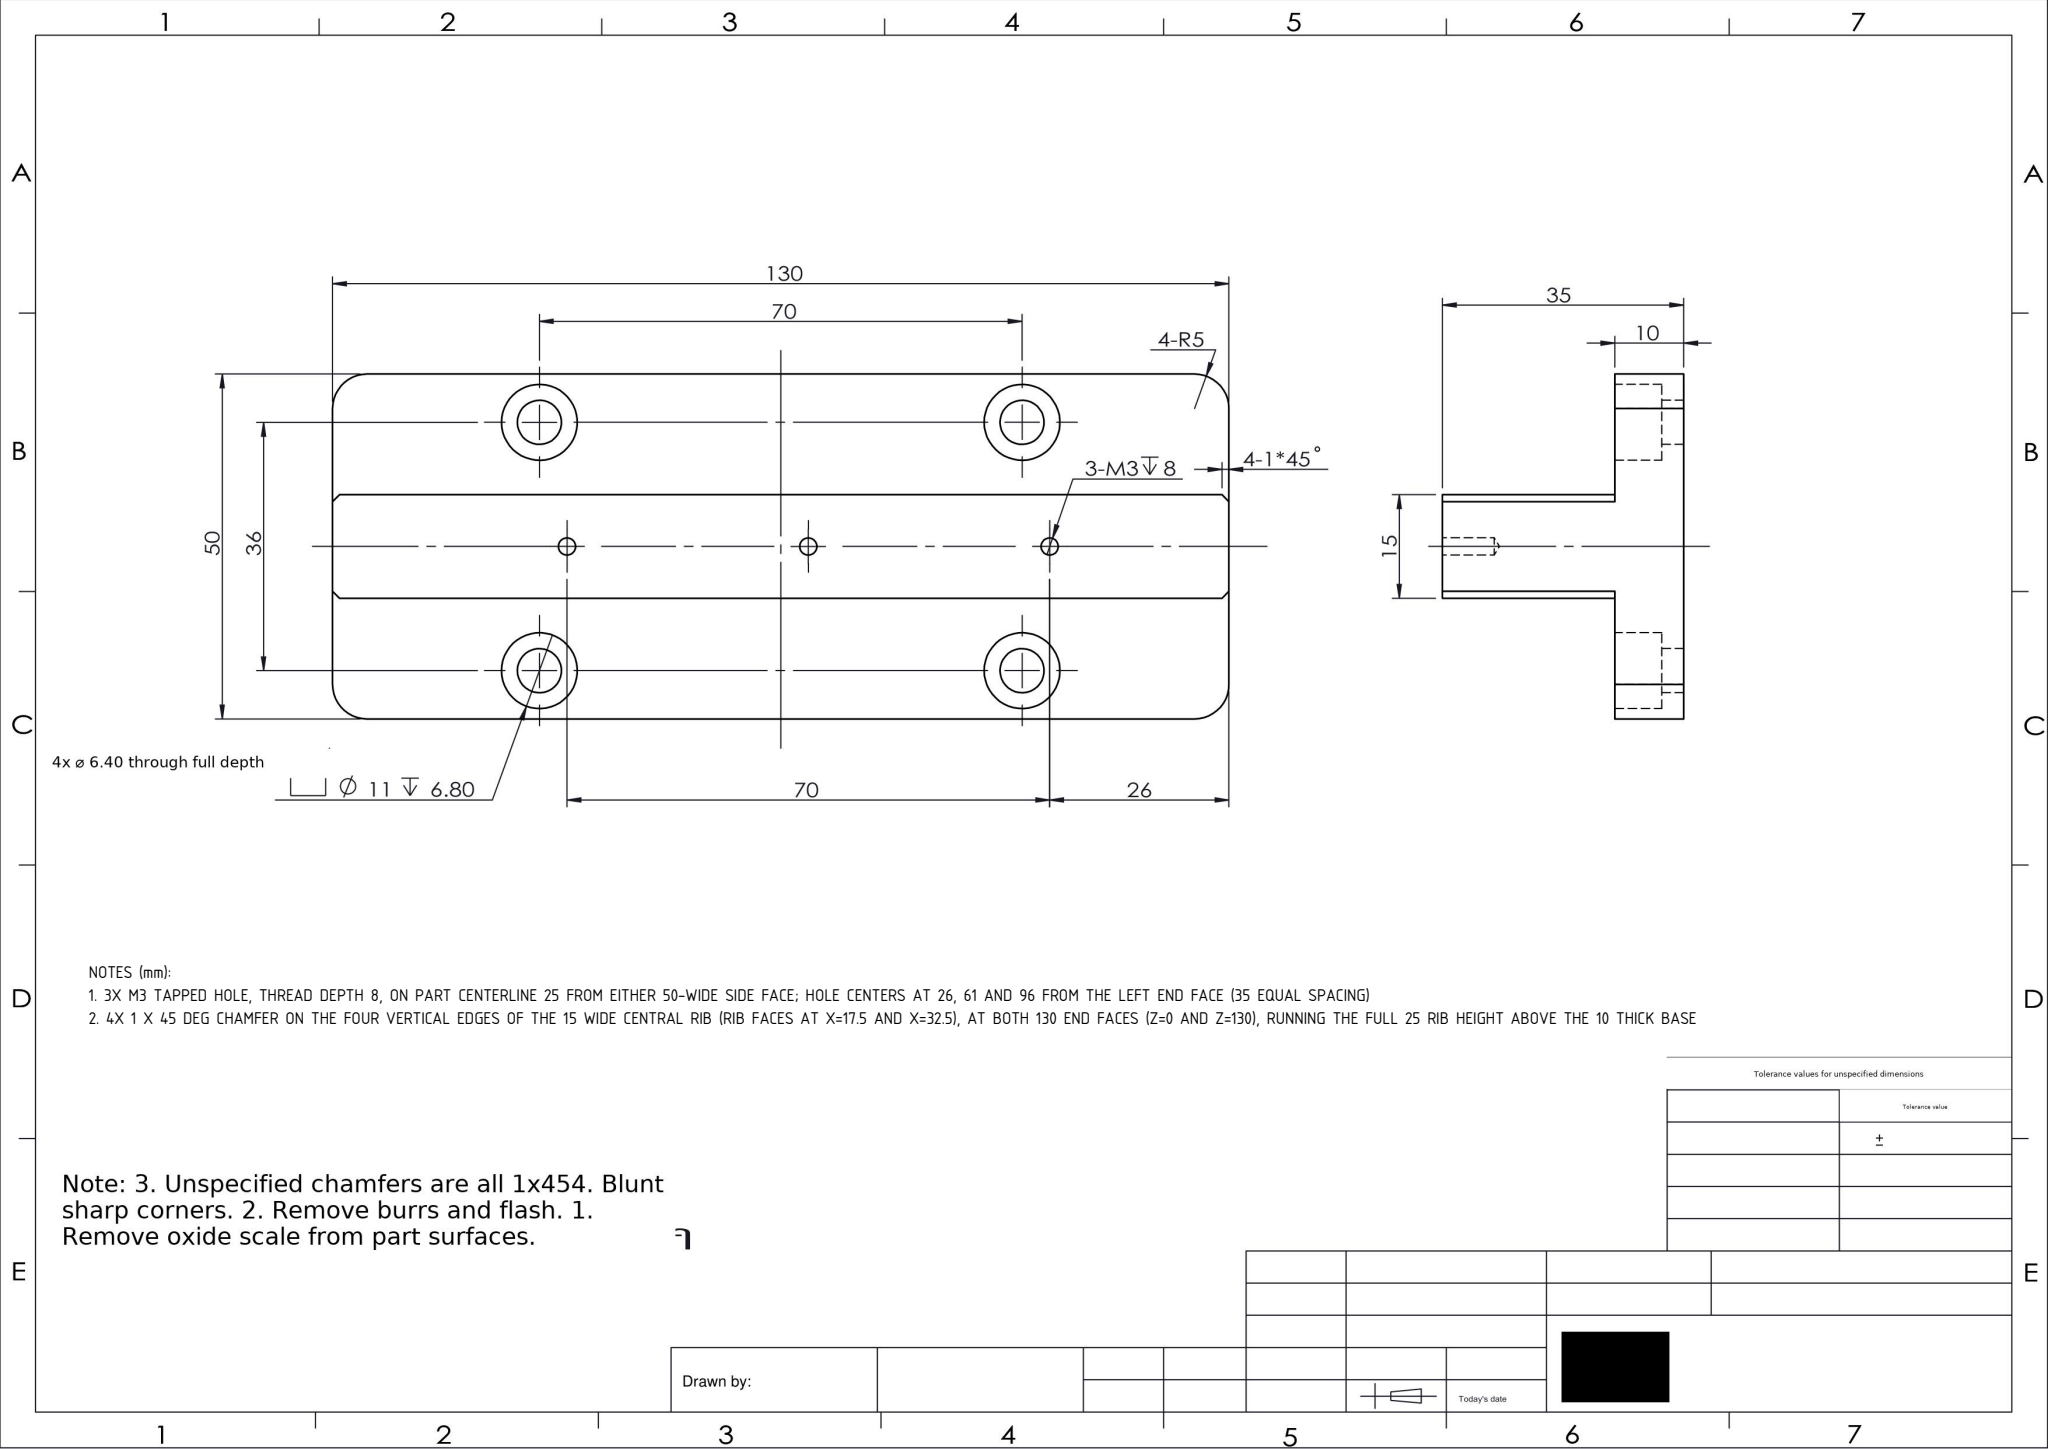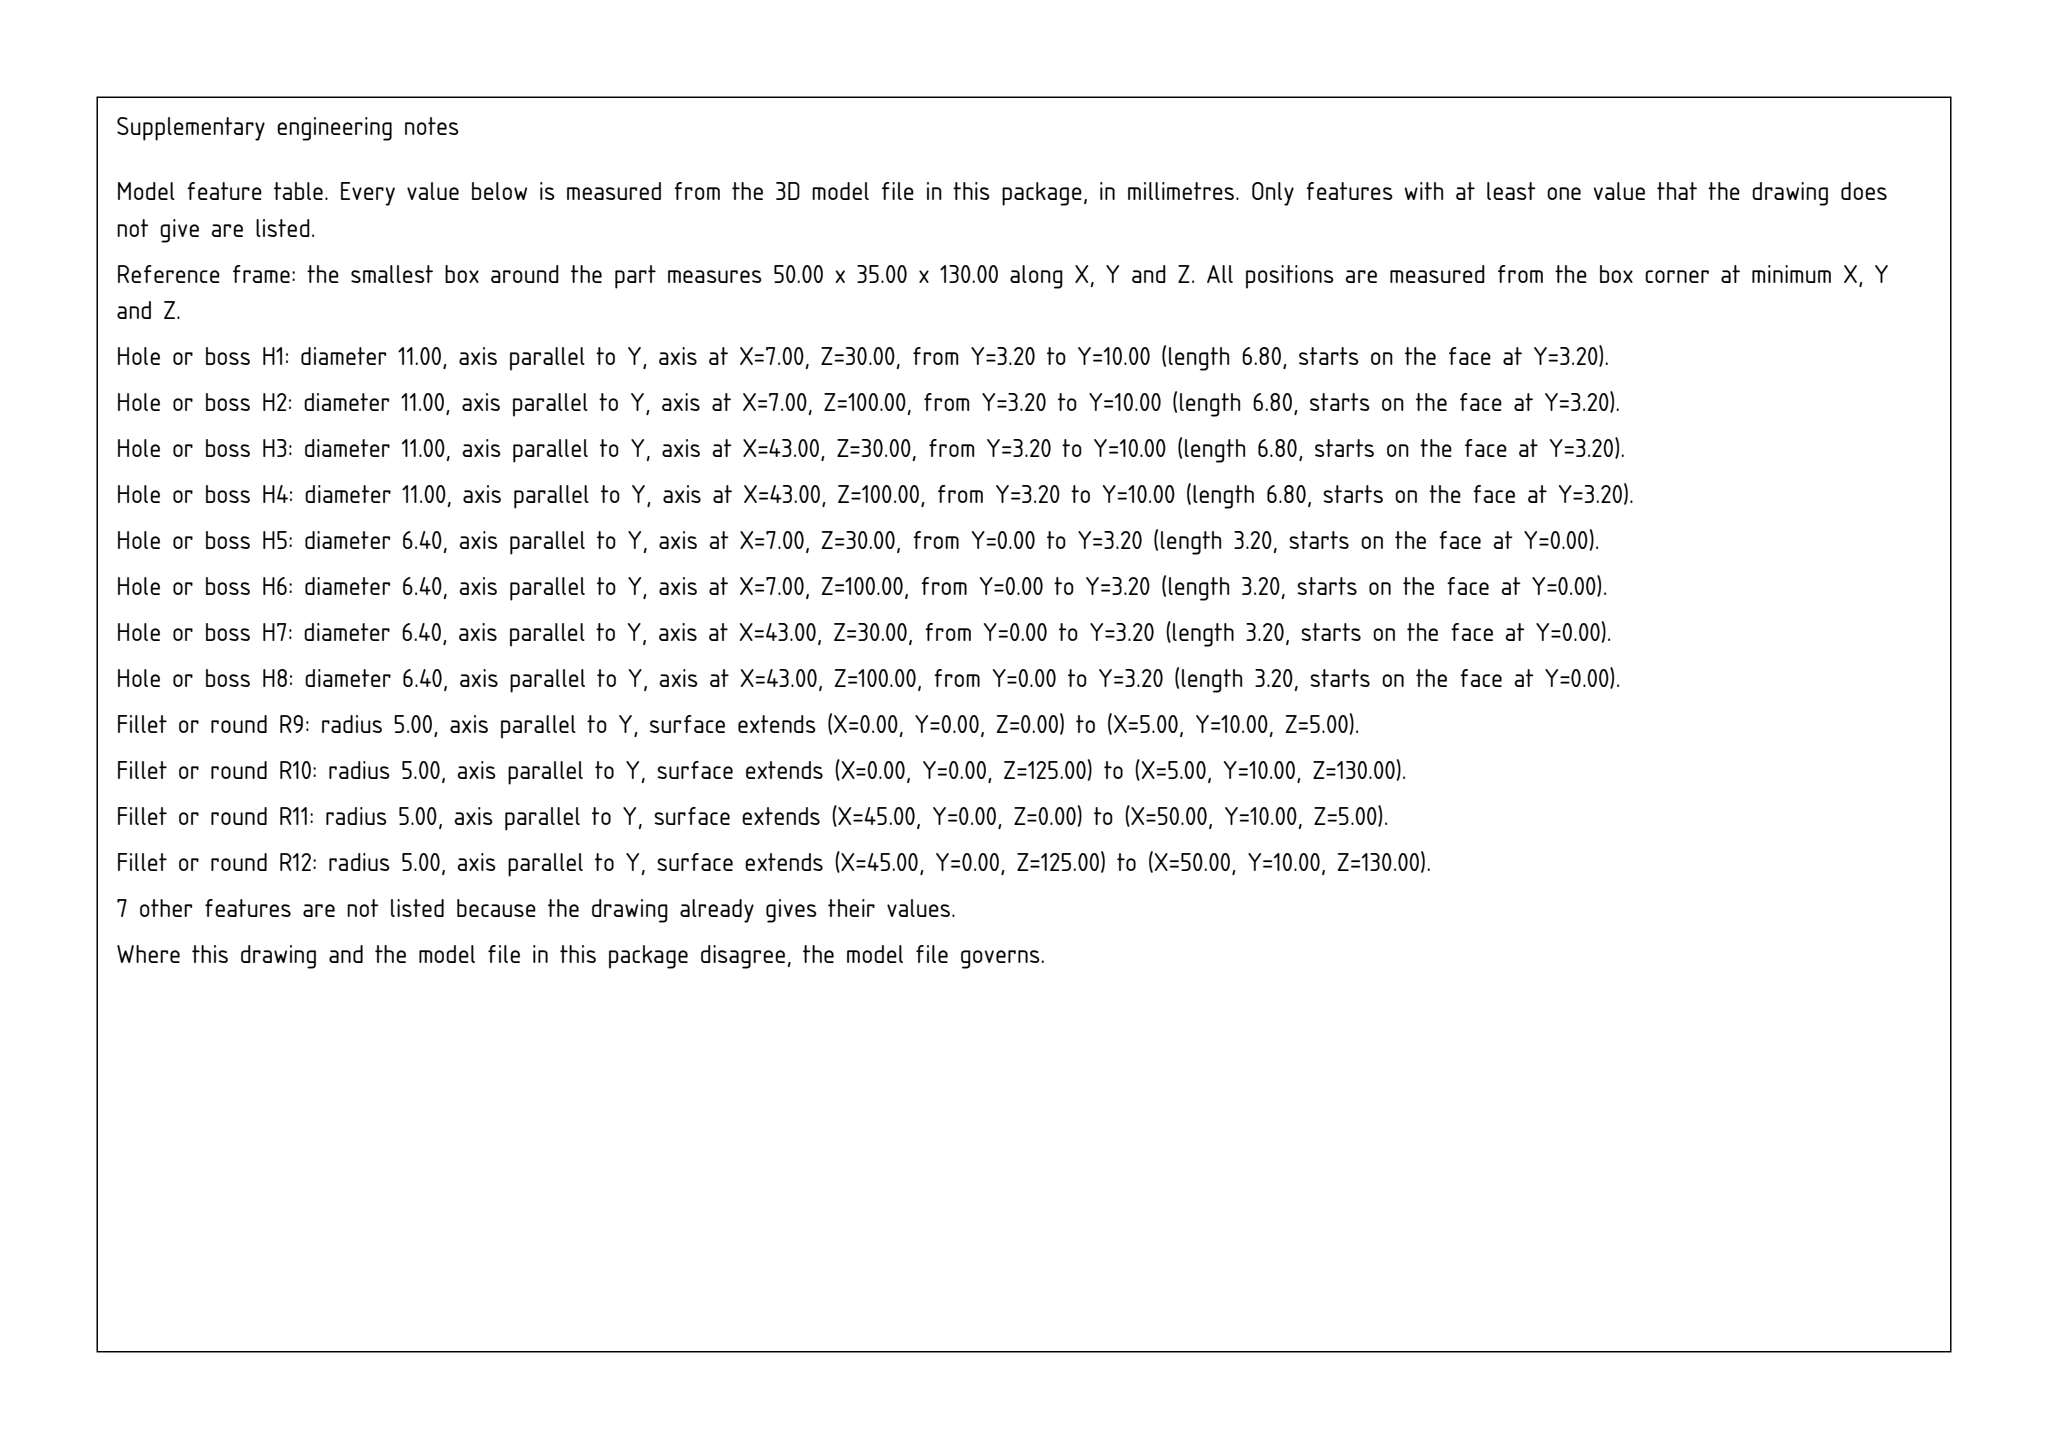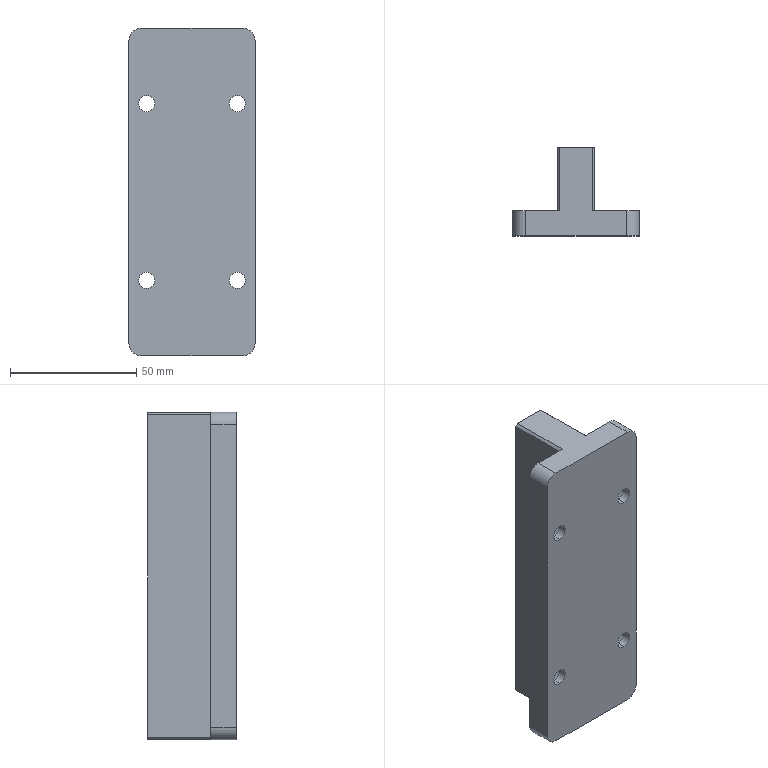Part | SolidWorks | mm | 1 solid | 50 faces | box 50 x 35 x 130 mm | volume 110375 mm3 | cylinder 26 | plane 18 | cone 6 | commonest cylinder face diameters 11 x8 6.4 x8 2.5 x6 10 x4
Drawing notes:
3X M3 TAPPED HOLE, THREAD DEPTH 8, ON PART CENTERLINE 25 FROM EITHER 50-WIDE SIDE FACE; HOLE CENTERS AT 26, 61 AND 96 FROM THE LEFT END FACE (35 EQUAL SPACING) | from the solid: cylinders: three 2.5 dia holes, axis y, at (x=25, z=26), (x=25, z=61), (x=25, z=96), from y=27.5 to y=35 (7.5 deep from top face of 35 tall rib)
4X 1 X 45 DEG CHAMFER ON THE FOUR VERTICAL EDGES OF THE 15 WIDE CENTRAL RIB (RIB FACES AT X=17.5 AND X=32.5), AT BOTH 130 END FACES (Z=0 AND Z=130), RUNNING THE FULL 25 RIB HEIGHT ABOVE THE 10 THICK BASE | from the solid: inclined_planes: four 45 deg faces, size 1 x 25 x 1, bbox_from [17.5,10,0], [17.5,10,129], [31.5,10,0], [31.5,10,129]
build123d program:
from build123d import *

# Parameters (mm, degrees)
BOSS_EXTRUDE1_DEPTH                                  = 130
HOLE_SIZE_ACCORDING_TO_THE_TYPE_OF_HEXAG_D           = 6.4
HOLE_SIZE_ACCORDING_TO_THE_TYPE_OF_HEXAG_CBORE_D     = 11
HOLE_SIZE_ACCORDING_TO_THE_TYPE_OF_HEXAG_CBORE_DEPTH = 6.8
LPATTERN1_COUNT                                      = 2
LPATTERN1_PITCH                                      = 70
FILLET1_R                                            = 5
CHAMFER2_SIZE                                        = 1
LPATTERN2_COUNT                                      = 3
LPATTERN2_PITCH                                      = 35


with BuildPart() as part:
    # Sketch1 → Boss-Extrude1 (new body)
    with BuildSketch(Plane.XY):
        Polygon((32.5, 10), (50, 10), (50, 0), (0, 0), (0, 10), (17.5, 10), (17.5, 35), (32.5, 35), align=None)
    extrude(amount=BOSS_EXTRUDE1_DEPTH)

    # Hole Size according to the type of Hexag (through all)
    with Locations(Plane(origin=(0, 10, 0), x_dir=(1, 0, 0), z_dir=(0, 1, 0))):
        with Locations((7, -30), (43, -30)):
            hole_size_according_to_the_type_of_hexag = CounterBoreHole(HOLE_SIZE_ACCORDING_TO_THE_TYPE_OF_HEXAG_D / 2, HOLE_SIZE_ACCORDING_TO_THE_TYPE_OF_HEXAG_CBORE_D / 2, HOLE_SIZE_ACCORDING_TO_THE_TYPE_OF_HEXAG_CBORE_DEPTH)

    # LPattern1: Hole Size according to the type of Hexag ×2
    with Locations(*[(0, 0, i * LPATTERN1_PITCH) for i in range(1, LPATTERN1_COUNT)]):
        add(hole_size_according_to_the_type_of_hexag, mode=Mode.SUBTRACT)

    # Fillet1
    fillet1_edges = [part.edges().sort_by_distance(p)[0] for p in [
        (50, 5, 130),
        (0, 5, 0),
        (0, 5, 130),
        (50, 5, 0),
    ]]
    fillet(fillet1_edges, radius=FILLET1_R)

    # Chamfer2
    chamfer2_edges = [part.edges().sort_by_distance(p)[0] for p in [
        (32.5, 22.5, 130),
        (17.5, 22.5, 130),
        (17.5, 22.5, 0),
        (32.5, 22.5, 0),
    ]]
    chamfer(chamfer2_edges, length=CHAMFER2_SIZE)

    # Sketch4 → M3 Tapped Hole1 (revolve, cut)
    with BuildSketch(Plane(origin=(25, 35, 26), x_dir=(0, 0, 1), z_dir=(1, 0, 0))):
        Polygon((0, 0), (0, 8.251), (1.25, 7.5), (1.25, 0), align=None)
    m3_tapped_hole1 = revolve(axis=Axis((25, 41.35, 26), (0, -1, 0)), mode=Mode.SUBTRACT)

    # LPattern2: M3 Tapped Hole1 ×3
    with Locations(*[(0, 0, i * LPATTERN2_PITCH) for i in range(1, LPATTERN2_COUNT)]):
        add(m3_tapped_hole1, mode=Mode.SUBTRACT)


solid = part.part